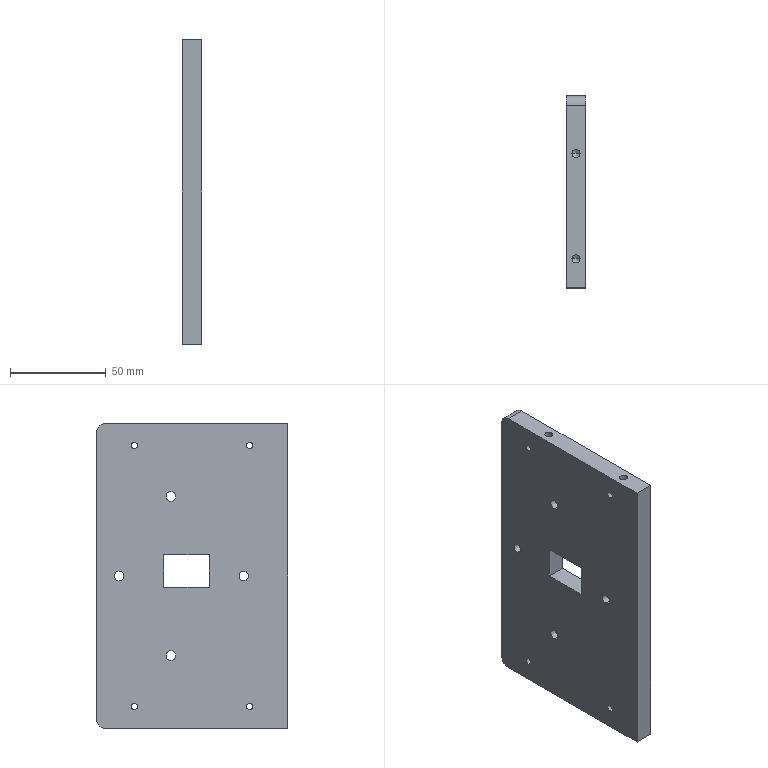Component | SolidWorks | FrameFrontPlate.1-1 | 1 solid | 44 faces | box 10 x 100 x 158.8 mm | volume 152841 mm3 | cylinder 26 | plane 10 | cone 8 | commonest cylinder face diameters 3.3 x8 4.2 x8 5 x8 10 x2
build123d program:
from build123d import *

# Parameters (mm, degrees)
BOSS_EXTRUDE1_DEPTH   = 10
M6_TAPPED_HOLE1_D     = 5
M6_TAPPED_HOLE1_DEPTH = 15
M6_TAPPED_HOLE1_TIP   = 1.502
M5_TAPPED_HOLE2_D     = 4.2
M5_TAPPED_HOLE2_DEPTH = 12.4
M5_TAPPED_HOLE2_TIP   = 1.262
M5_TAPPED_HOLE3_D     = 4.2
M5_TAPPED_HOLE3_DEPTH = 12.4
M5_TAPPED_HOLE3_TIP   = 1.262
LPATTERN1_COUNT       = 2
LPATTERN1_PITCH       = 136
LPATTERN1_COUNT_DIR2  = 2
LPATTERN1_PITCH_DIR2  = 60
SKETCH1_W             = 16.9
SKETCH1_H             = 23.75
CUT_EXTRUDE1_DEPTH    = 25


with BuildPart() as part:
    # Sketch1_2 → Boss-Extrude1 (new body)
    with BuildSketch(Plane.XY):
        with BuildLine():
            Line((-74.4, 100), (74.4, 100))
            ThreePointArc((74.4, 100), (77.936, 98.536), (79.4, 95))
            Line((79.4, 95), (79.4, 0))
            Line((79.4, 0), (-79.4, 0))
            Line((-79.4, 0), (-79.4, 95))
            ThreePointArc((-79.4, 95), (-77.936, 98.536), (-74.4, 100))
        make_face()
    extrude(amount=BOSS_EXTRUDE1_DEPTH)

    # M6 Tapped Hole1
    with Locations(Plane.XY.offset(10)):
        with Locations((0, 88), (0, 23), (-41.5, 61), (41.5, 61)):
            Hole(M6_TAPPED_HOLE1_D / 2, depth=M6_TAPPED_HOLE1_DEPTH)
            with Locations((0, 0, -(M6_TAPPED_HOLE1_DEPTH + M6_TAPPED_HOLE1_TIP / 2))):  # 118° drill point
                Cone(0, M6_TAPPED_HOLE1_D / 2, M6_TAPPED_HOLE1_TIP, mode=Mode.SUBTRACT)

    # M5 Tapped Hole2
    with Locations(Plane(origin=(79.4, 0, 0), x_dir=(0, 0, -1), z_dir=(1, 0, 0))):
        with Locations((-5, 15), (-5, 70)):
            Hole(M5_TAPPED_HOLE2_D / 2, depth=M5_TAPPED_HOLE2_DEPTH)
            with Locations((0, 0, -(M5_TAPPED_HOLE2_DEPTH + M5_TAPPED_HOLE2_TIP / 2))):  # 118° drill point
                Cone(0, M5_TAPPED_HOLE2_D / 2, M5_TAPPED_HOLE2_TIP, mode=Mode.SUBTRACT)

    # M5 Tapped Hole3
    with Locations(Plane.ZY.offset(79.4)):
        with Locations((5, 70), (5, 15)):
            Hole(M5_TAPPED_HOLE3_D / 2, depth=M5_TAPPED_HOLE3_DEPTH)
            with Locations((0, 0, -(M5_TAPPED_HOLE3_DEPTH + M5_TAPPED_HOLE3_TIP / 2))):  # 118° drill point
                Cone(0, M5_TAPPED_HOLE3_D / 2, M5_TAPPED_HOLE3_TIP, mode=Mode.SUBTRACT)

    # Sketch9 → M4 Tapped Hole1 (revolve, cut)
    with BuildSketch(Plane(origin=(-68, 80, 10), x_dir=(0, -1, 0), z_dir=(1, 0, 0))):
        Polygon((0, 0), (0, 11.091), (1.65, 10.1), (1.65, 0), align=None)
    m4_tapped_hole1 = revolve(axis=Axis((-68, 80, 16.35), (0, 0, -1)), mode=Mode.SUBTRACT)

    # LPattern1: M4 Tapped Hole1 2 × 2
    with Locations(*[(i * LPATTERN1_PITCH, -j * LPATTERN1_PITCH_DIR2, 0) for i in range(LPATTERN1_COUNT) for j in range(LPATTERN1_COUNT_DIR2) if (i, j) != (0, 0)]):
        add(m4_tapped_hole1, mode=Mode.SUBTRACT)

    # Sketch1 → Cut-Extrude1 (cut, symmetric)
    with BuildSketch(Plane.XY):
        with Locations((2.6, 52.875)):
            Rectangle(SKETCH1_W, SKETCH1_H)
    extrude(amount=CUT_EXTRUDE1_DEPTH, both=True, mode=Mode.SUBTRACT)


solid = part.part

# Placed as in the assembly
solid = solid.moved(Location((-45.5, 268, 0), (0, -90, 0)))